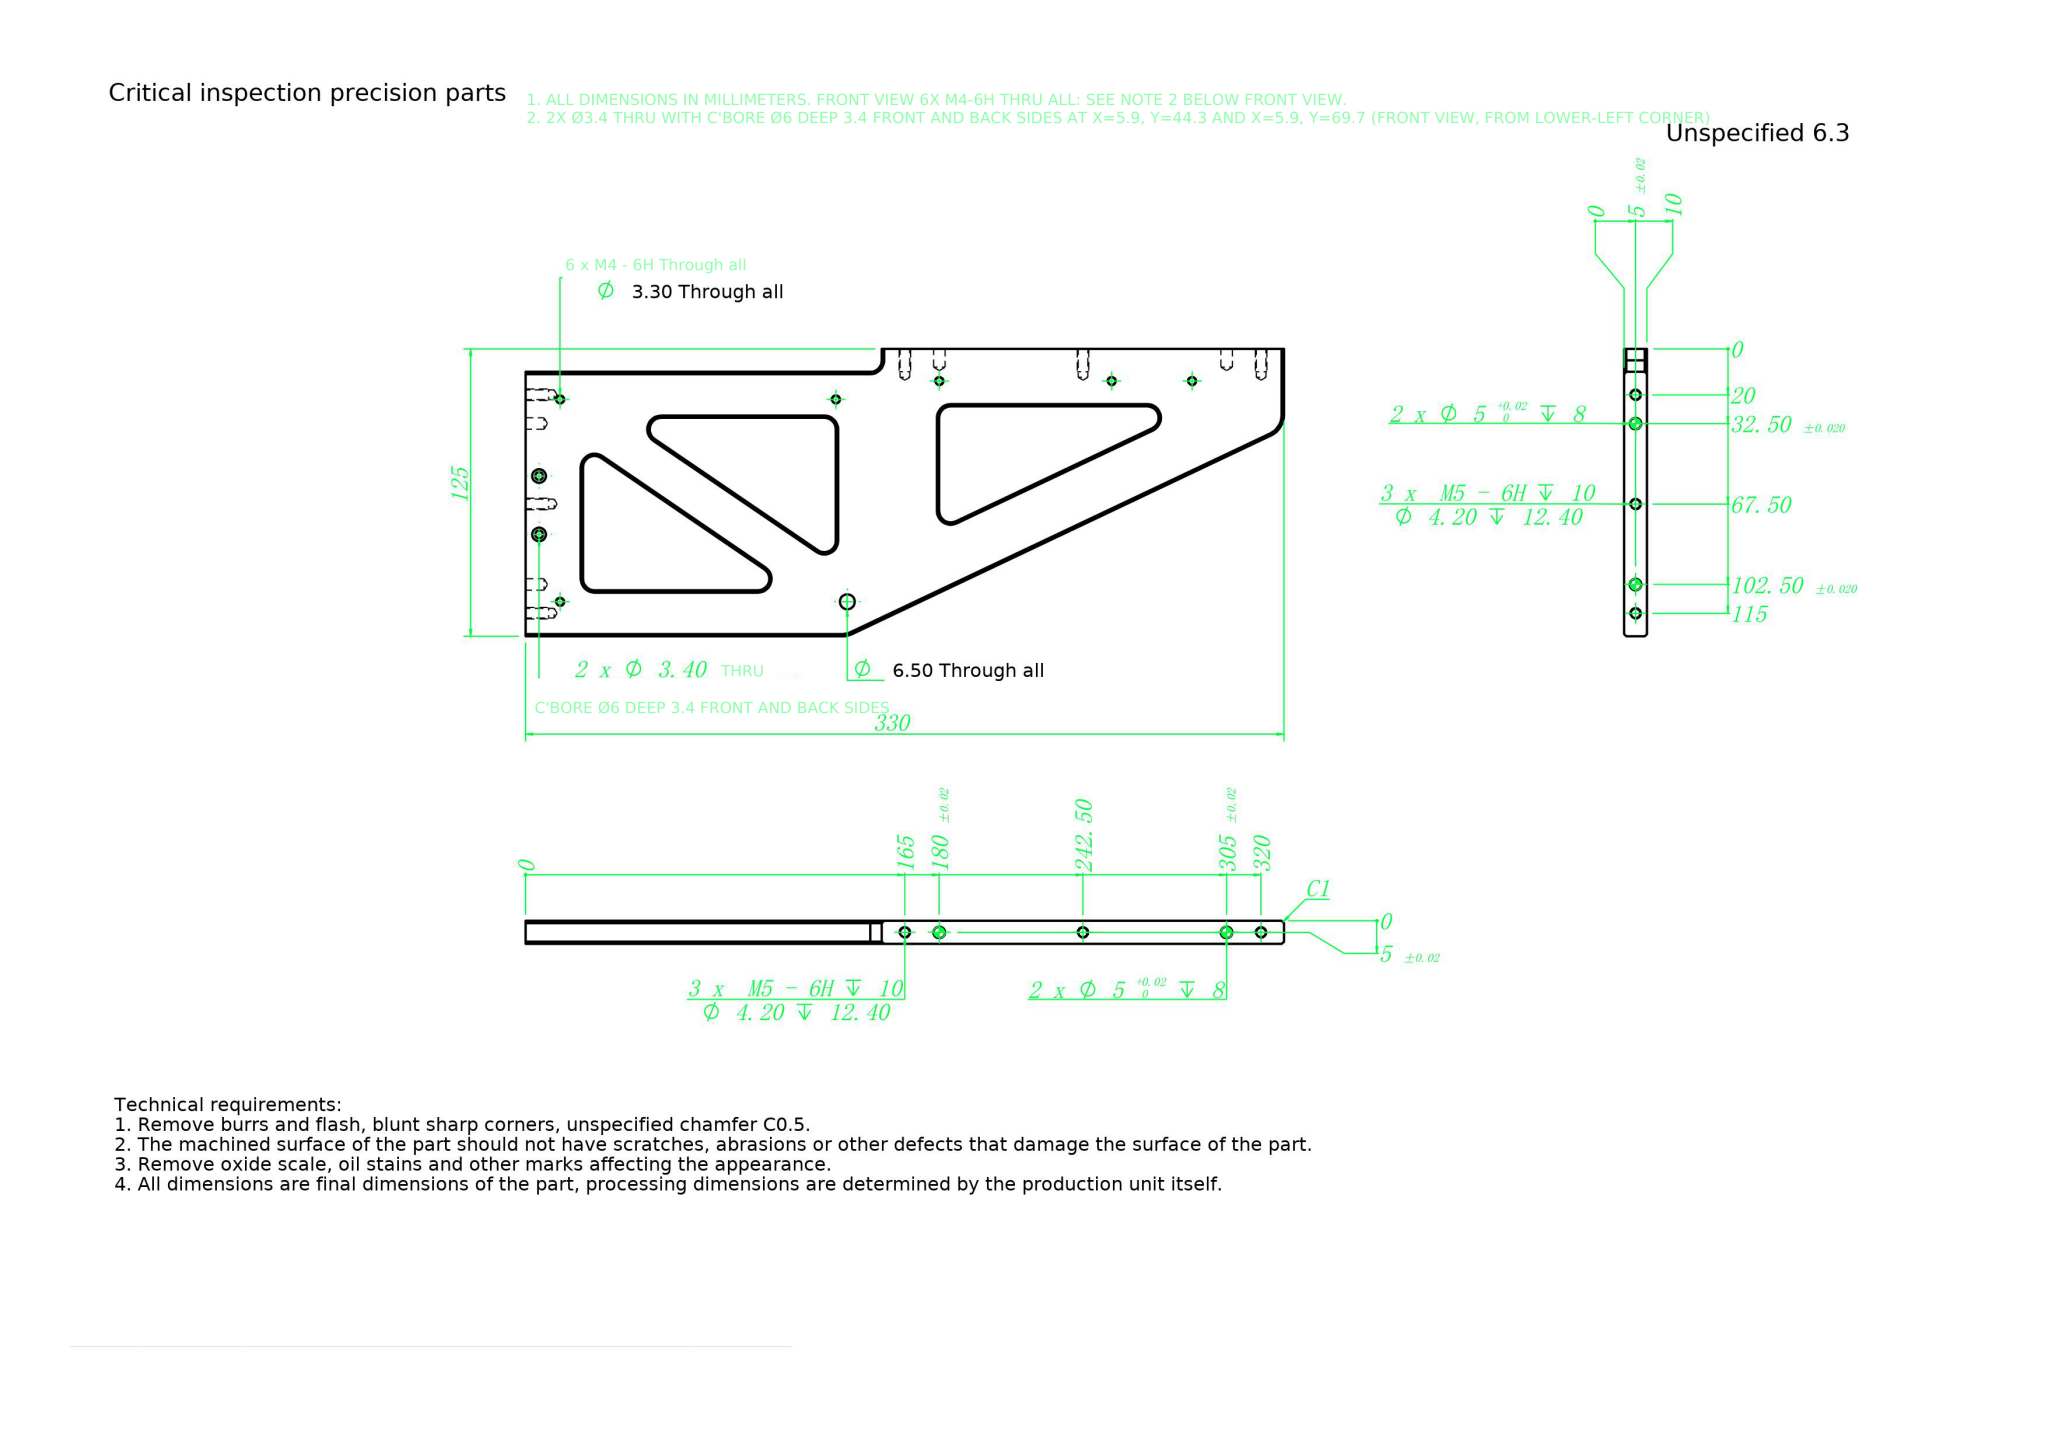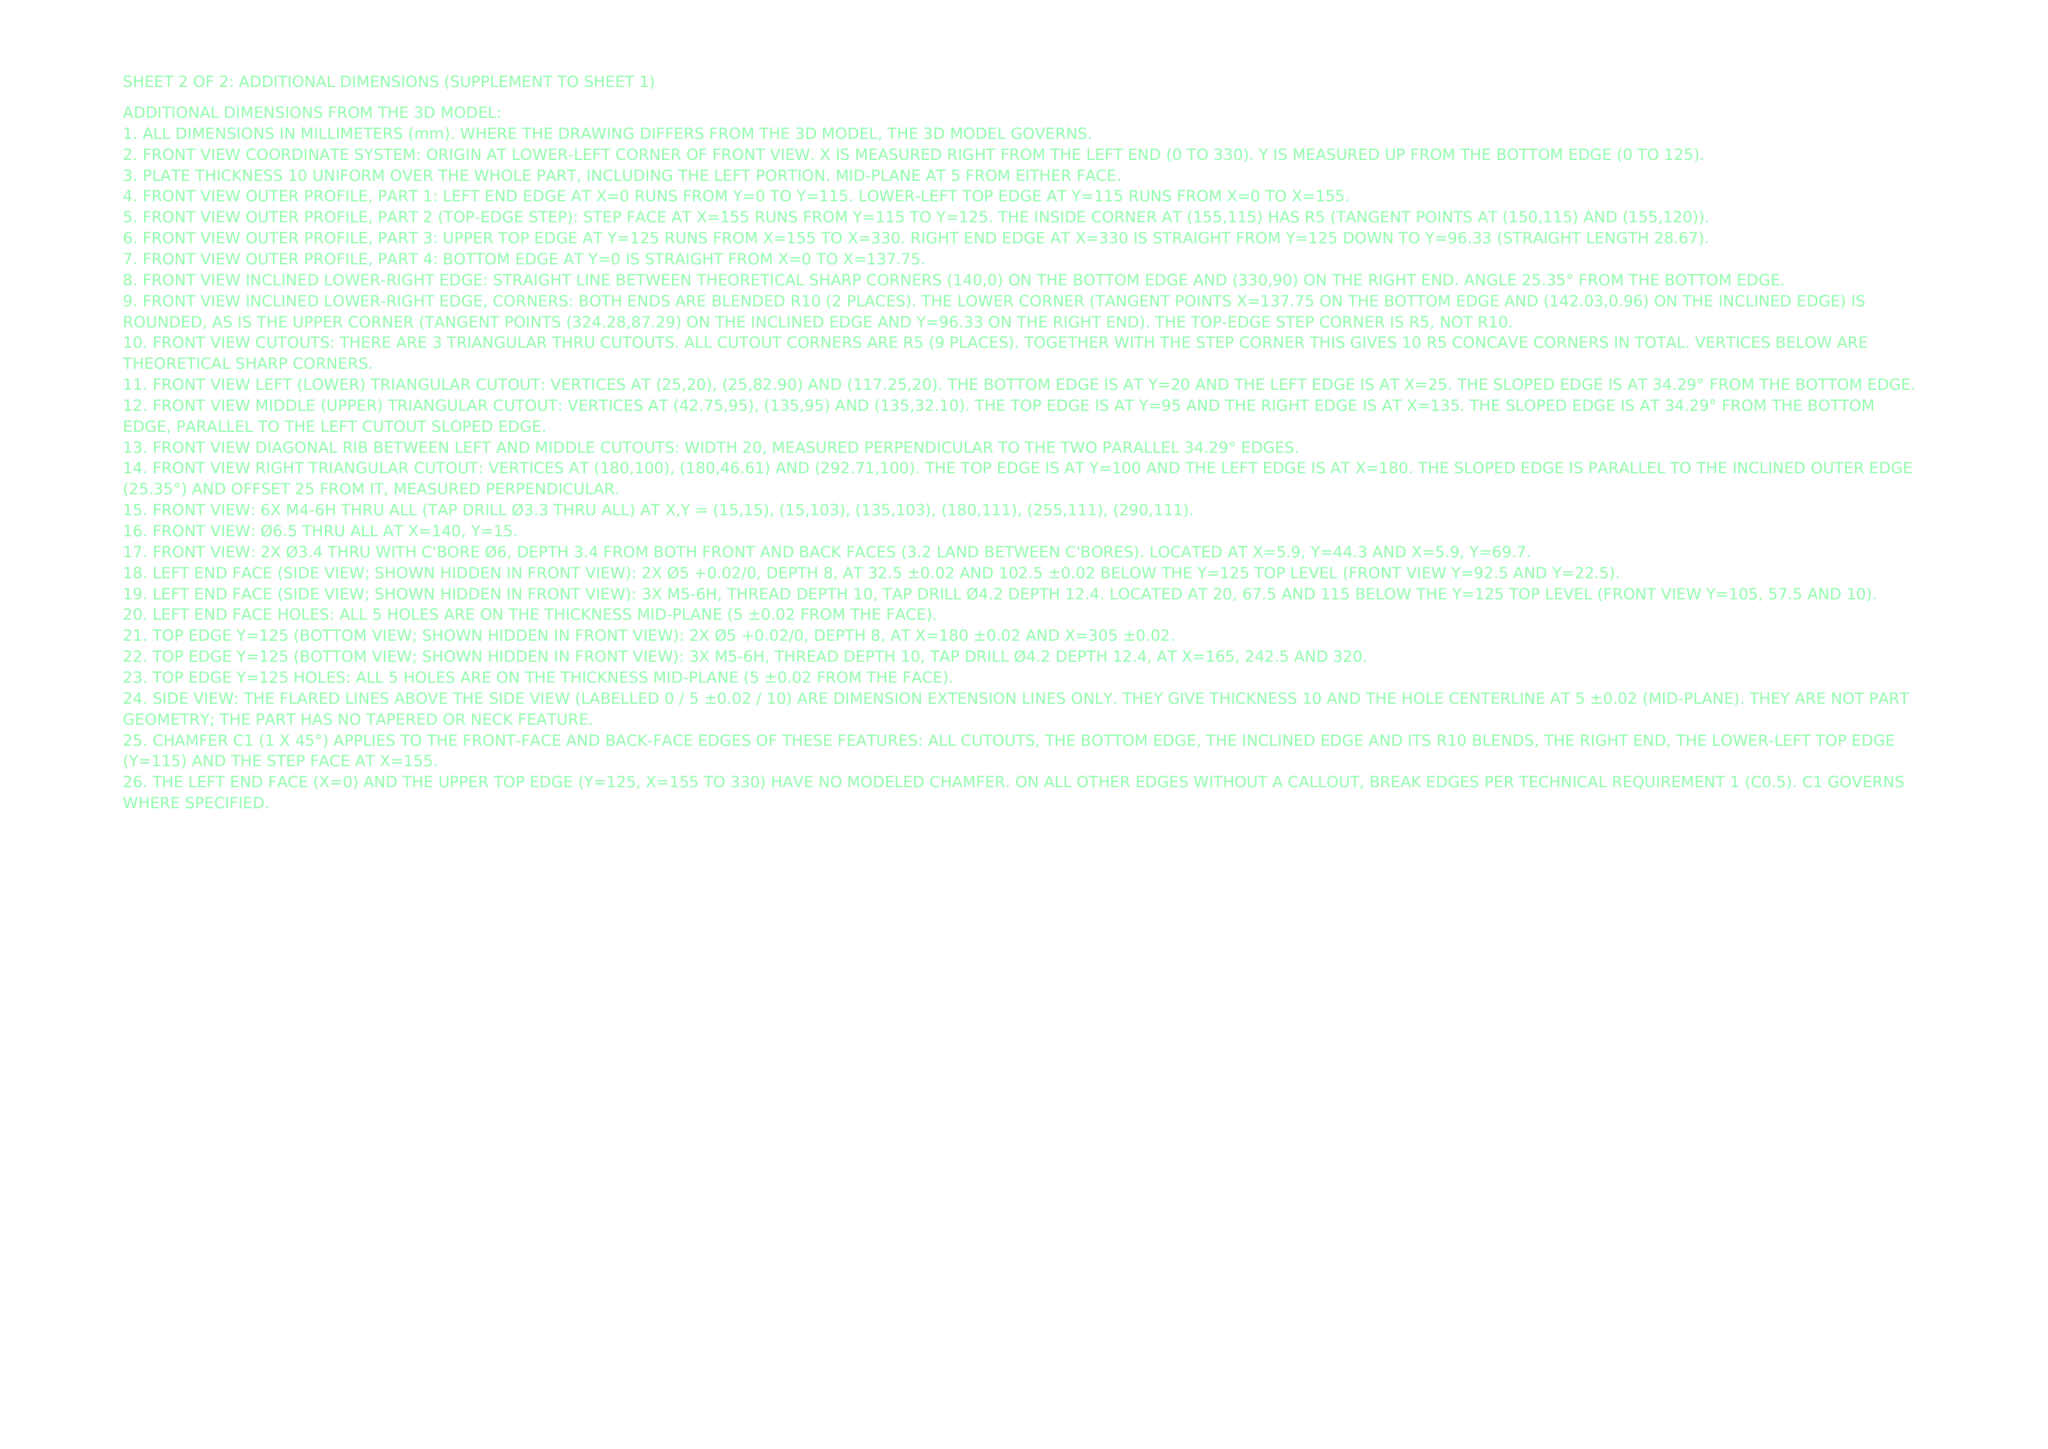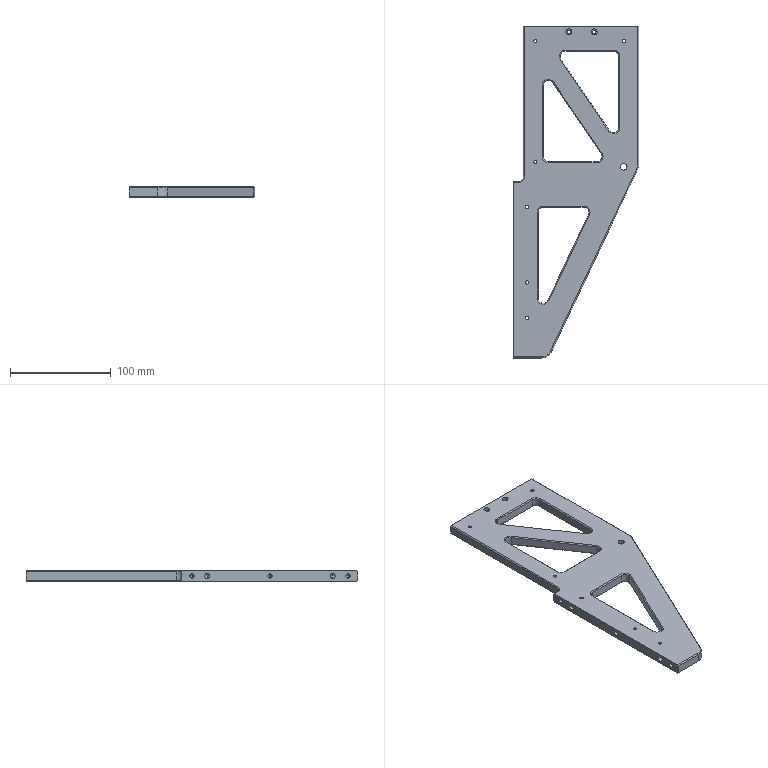Part | NX | mm | 1 solid | 157 faces | box 125 x 330 x 10 mm | volume 221540 mm3 | cylinder 60 | plane 50 | cone 47 | commonest cylinder face diameters 3.3 x12 4.2 x12 10 x12 6 x8 5 x8 3.4 x4 6.5 x2 20 x2